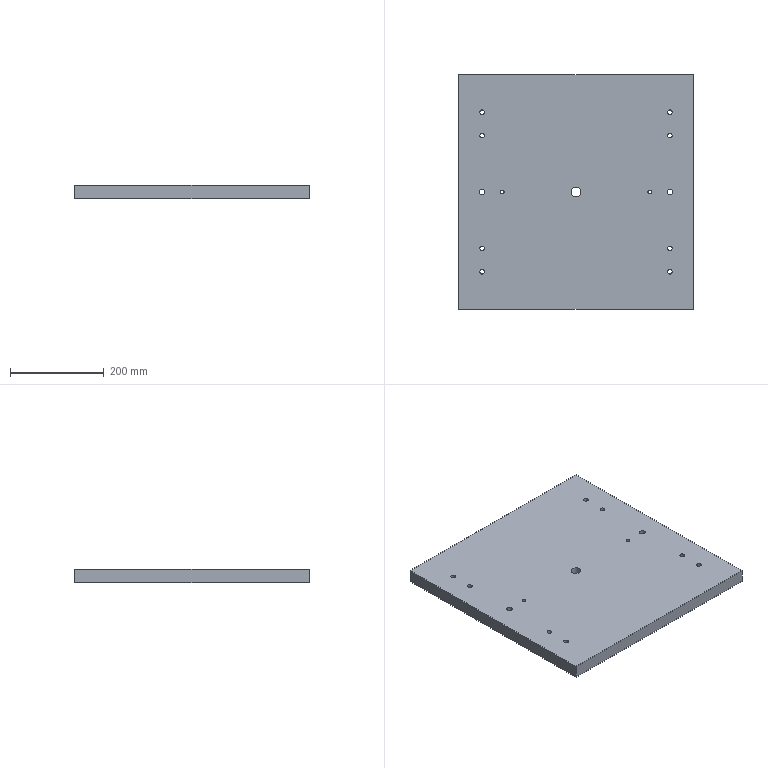Component | NX | DIE_FIX_PLATE | 1 solid | 27 faces | volume 6964024 mm3 | cylinder 13 | cone 8 | plane 6 | commonest cylinder face diameters 10 x4 9.732 x4 12 x2 8 x2 21 x1